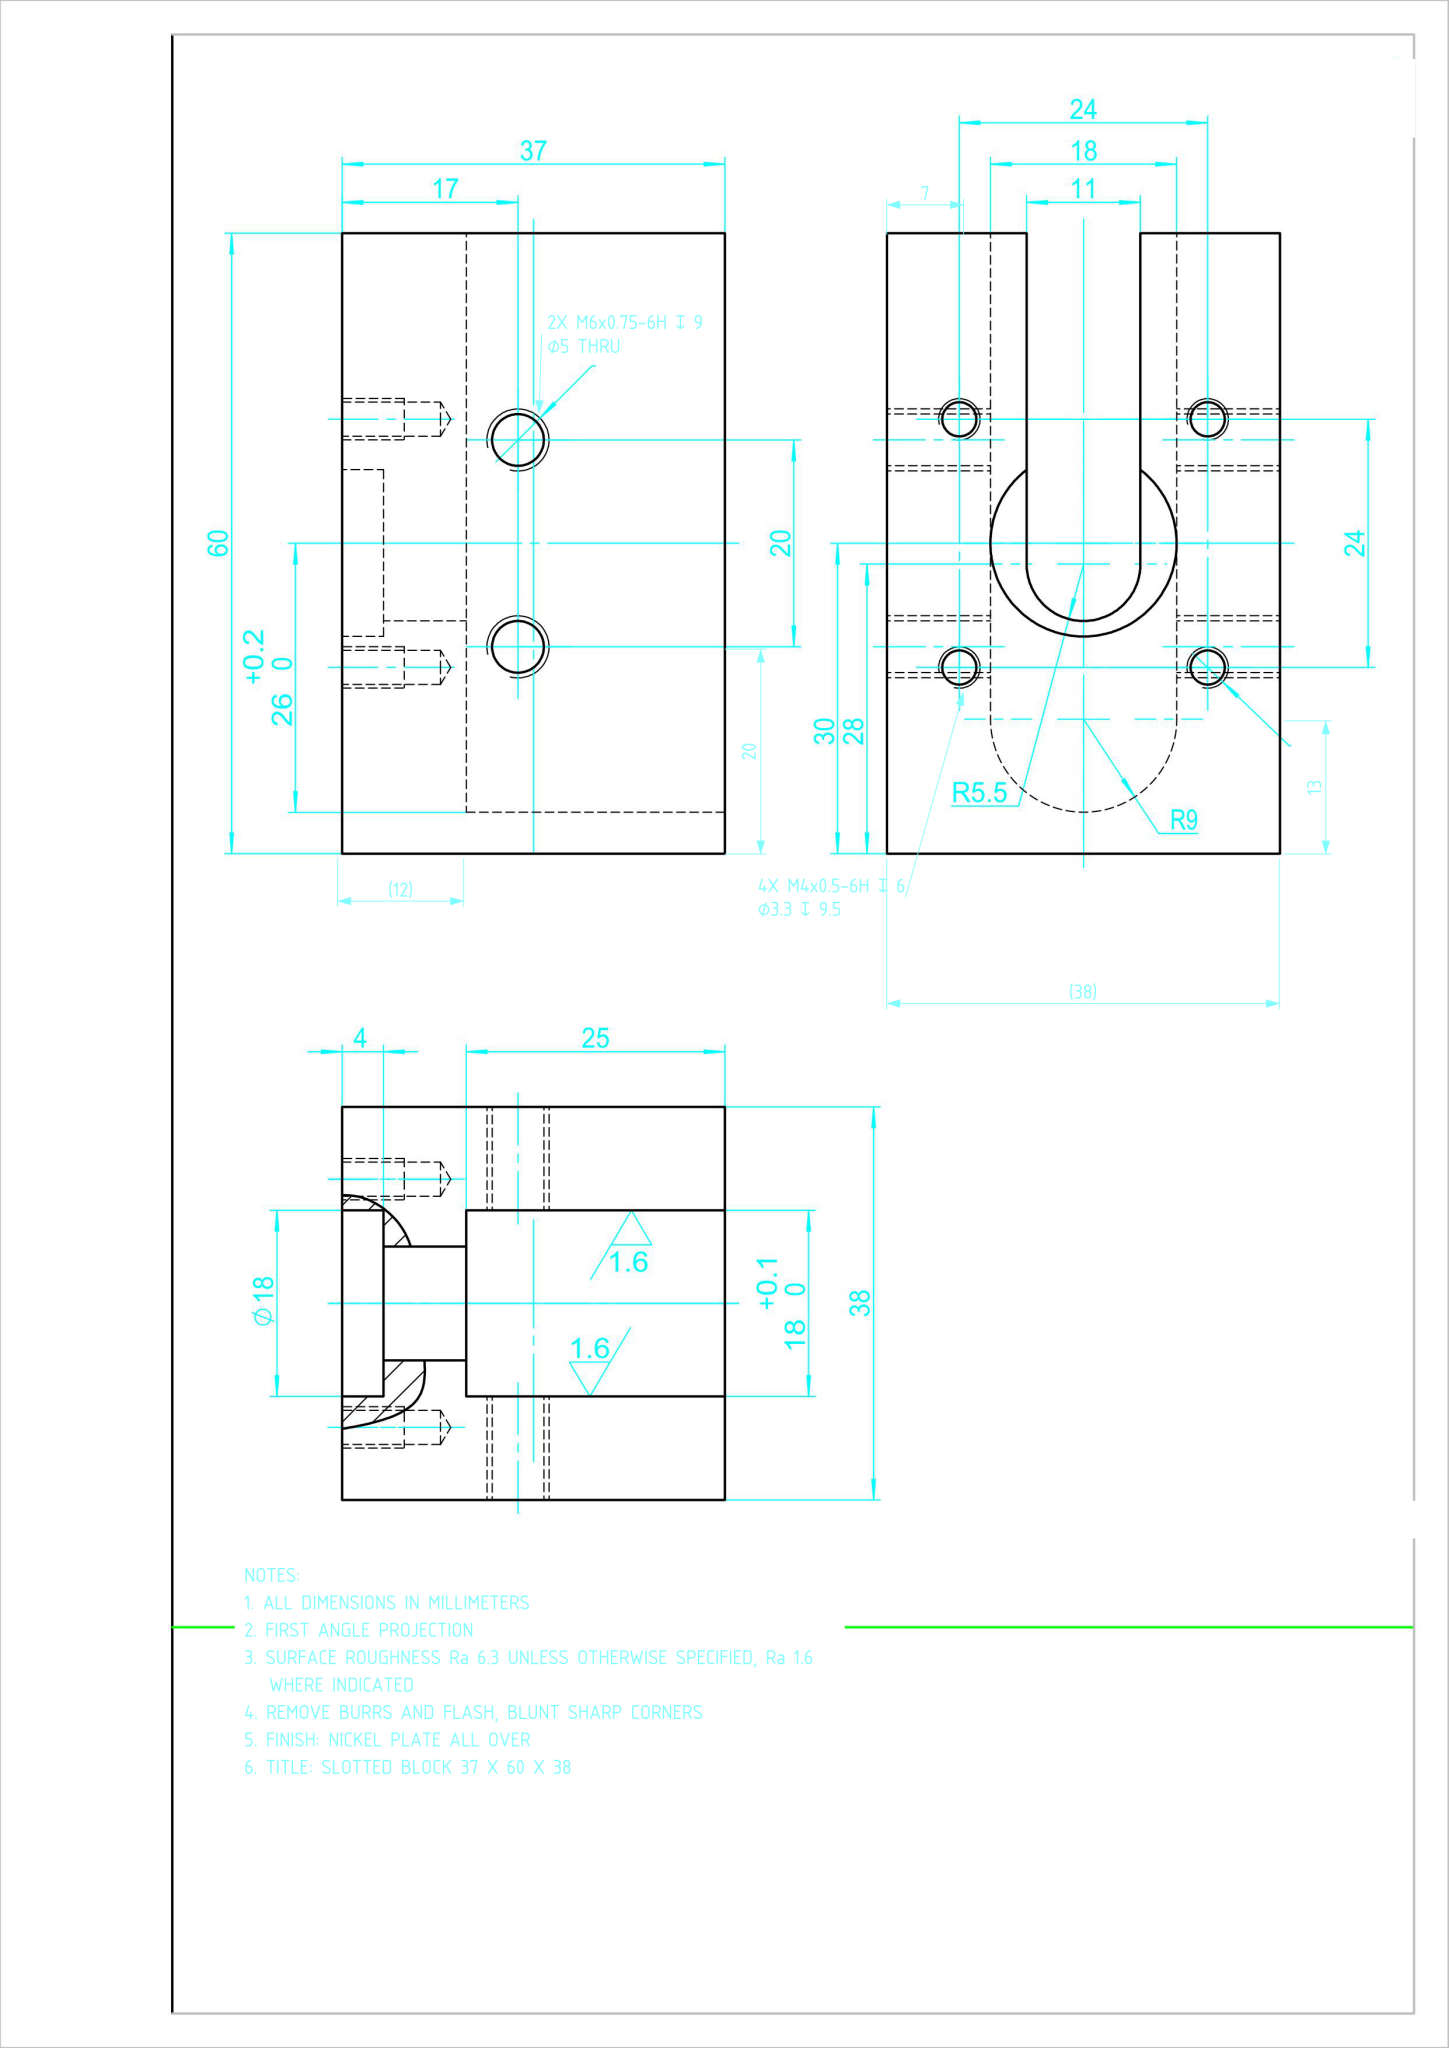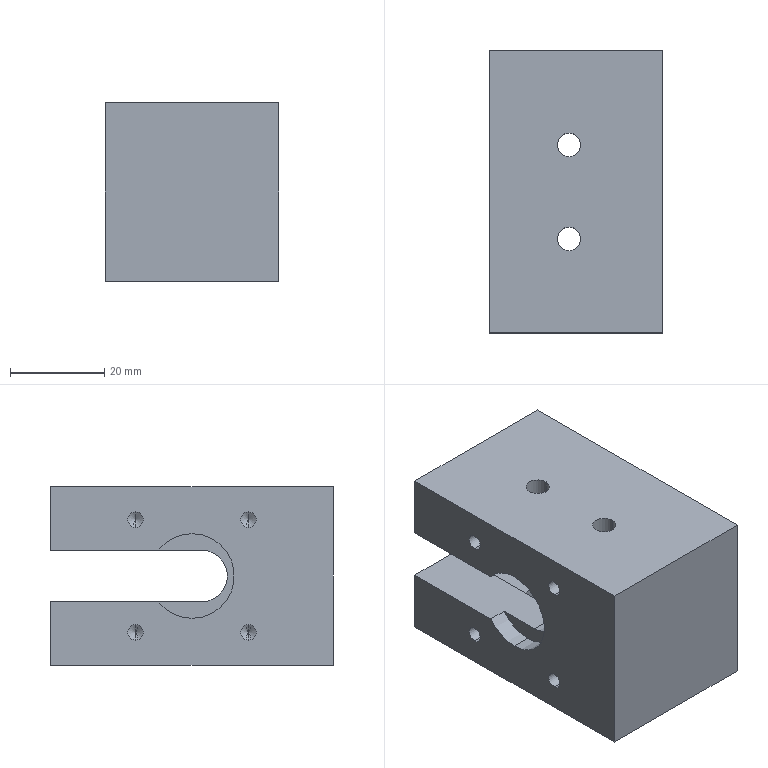Part | NX | mm | 1 solid | 42 faces | box 37 x 60 x 38 mm | volume 53743 mm3 | cylinder 21 | plane 13 | cone 8 | commonest cylinder face diameters 3.3 x8 5 x8 18 x4 11 x1